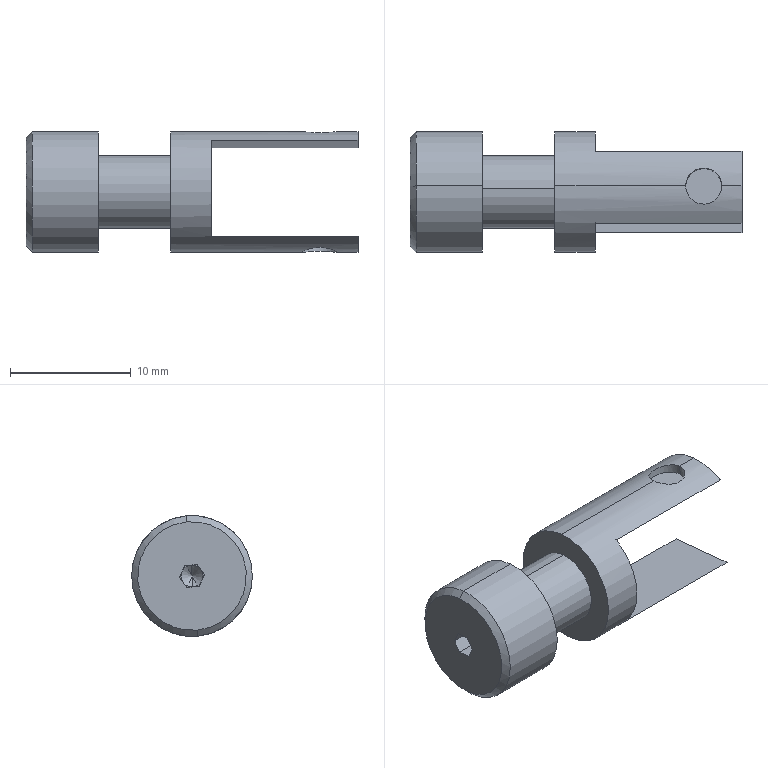Component | SolidWorks | PHSLN125-1_PHSLN125_SCREW_SCREW-1 | 1 solid | 36 faces | box 27.5 x 10 x 10 mm | volume 982 mm3 | plane 22 | cylinder 10 | cone 4 | commonest cylinder face diameters 3 x4 10 x4 6 x2
build123d program:
from build123d import *

# Parameters (mm, degrees)
CUT_EXTRUDE1_DEPTH      = 5
CUT_EXTRUDE1_DEPTH_BACK = 5
SKETCH2_W               = 12.167
SKETCH2_H               = 8
SKETCH3_R               = 1.5
CUT_EXTRUDE2_DEPTH      = 0.8
CUT_EXTRUDE3_START      = 0.8
SKETCH4_R               = 1.5
CUT_EXTRUDE3_DEPTH      = 0.8
CUT_EXTRUDE4_DEPTH      = 1.8


with BuildPart() as part:
    # Sketch1 → Revolve1 (revolve)
    with BuildSketch(Plane.XY, mode=Mode.PRIVATE) as revolve1_sk:
        Polygon((-18, 0), (-18, 4.5), (-17.5, 5), (-12, 5), (-12, 3), (-6, 3), (-6, 5), (9.5, 5), (9.5, 0), align=None)
    revolve(revolve1_sk.sketch.rotate(Axis((9.5, 0, 0), (-1, 0, 0)), 270), axis=Axis((9.5, 0, 0), (-1, 0, 0)))

    # Sketch2 → Cut-Extrude1 (cut, two sides: drawn at the far end of the back side and taken through both)
    with BuildSketch(Plane(origin=(0, 0, 0), x_dir=(1, 0, 0), z_dir=(0, 1, 0)).offset(-CUT_EXTRUDE1_DEPTH_BACK)):
        with Locations((3.417, 0)):
            Rectangle(SKETCH2_W, SKETCH2_H)
    extrude(amount=CUT_EXTRUDE1_DEPTH + CUT_EXTRUDE1_DEPTH_BACK, mode=Mode.SUBTRACT)

    # Sketch3 → Cut-Extrude2 (cut)
    with BuildSketch(Plane.XY.offset(5)):
        with Locations((6.333, 0)):
            Circle(SKETCH3_R)
    extrude(amount=-CUT_EXTRUDE2_DEPTH, mode=Mode.SUBTRACT)

    # Sketch4 → Cut-Extrude3 (cut)
    with BuildSketch(Plane.XY.offset(-5).offset(CUT_EXTRUDE3_START)):
        with Locations((6.333, 0)):
            Circle(SKETCH4_R)
    extrude(amount=-CUT_EXTRUDE3_DEPTH, mode=Mode.SUBTRACT)

    # Sketch5 → Cut-Extrude4 (cut)
    with BuildSketch(Plane(origin=(-18, 0, 0), x_dir=(0, 0, -1), z_dir=(1, 0, 0))):
        Polygon((-0.9, 0.5196), (-0.9, -0.5196), (0, -1.039), (0.9, -0.5196), (0.9, 0.5196), (0, 1.039), align=None)
    extrude(amount=CUT_EXTRUDE4_DEPTH, mode=Mode.SUBTRACT)

    # Sketch6 → Cut-Revolve1 (revolve, cut)
    with BuildSketch(Plane.XY, mode=Mode.PRIVATE) as cut_revolve1_sk:
        Polygon((-16.2, 0), (-16.2, 0.9), (-15.3, 0), align=None)
    revolve(cut_revolve1_sk.sketch.rotate(Axis((-15.3, 0, 0), (-1, 0, 0)), 270), axis=Axis((-15.3, 0, 0), (-1, 0, 0)), mode=Mode.SUBTRACT)


solid = part.part

# Placed as in the assembly
solid = solid.moved(Location((601.5, 80.244, -5.079), (174.228, 0, 0)))